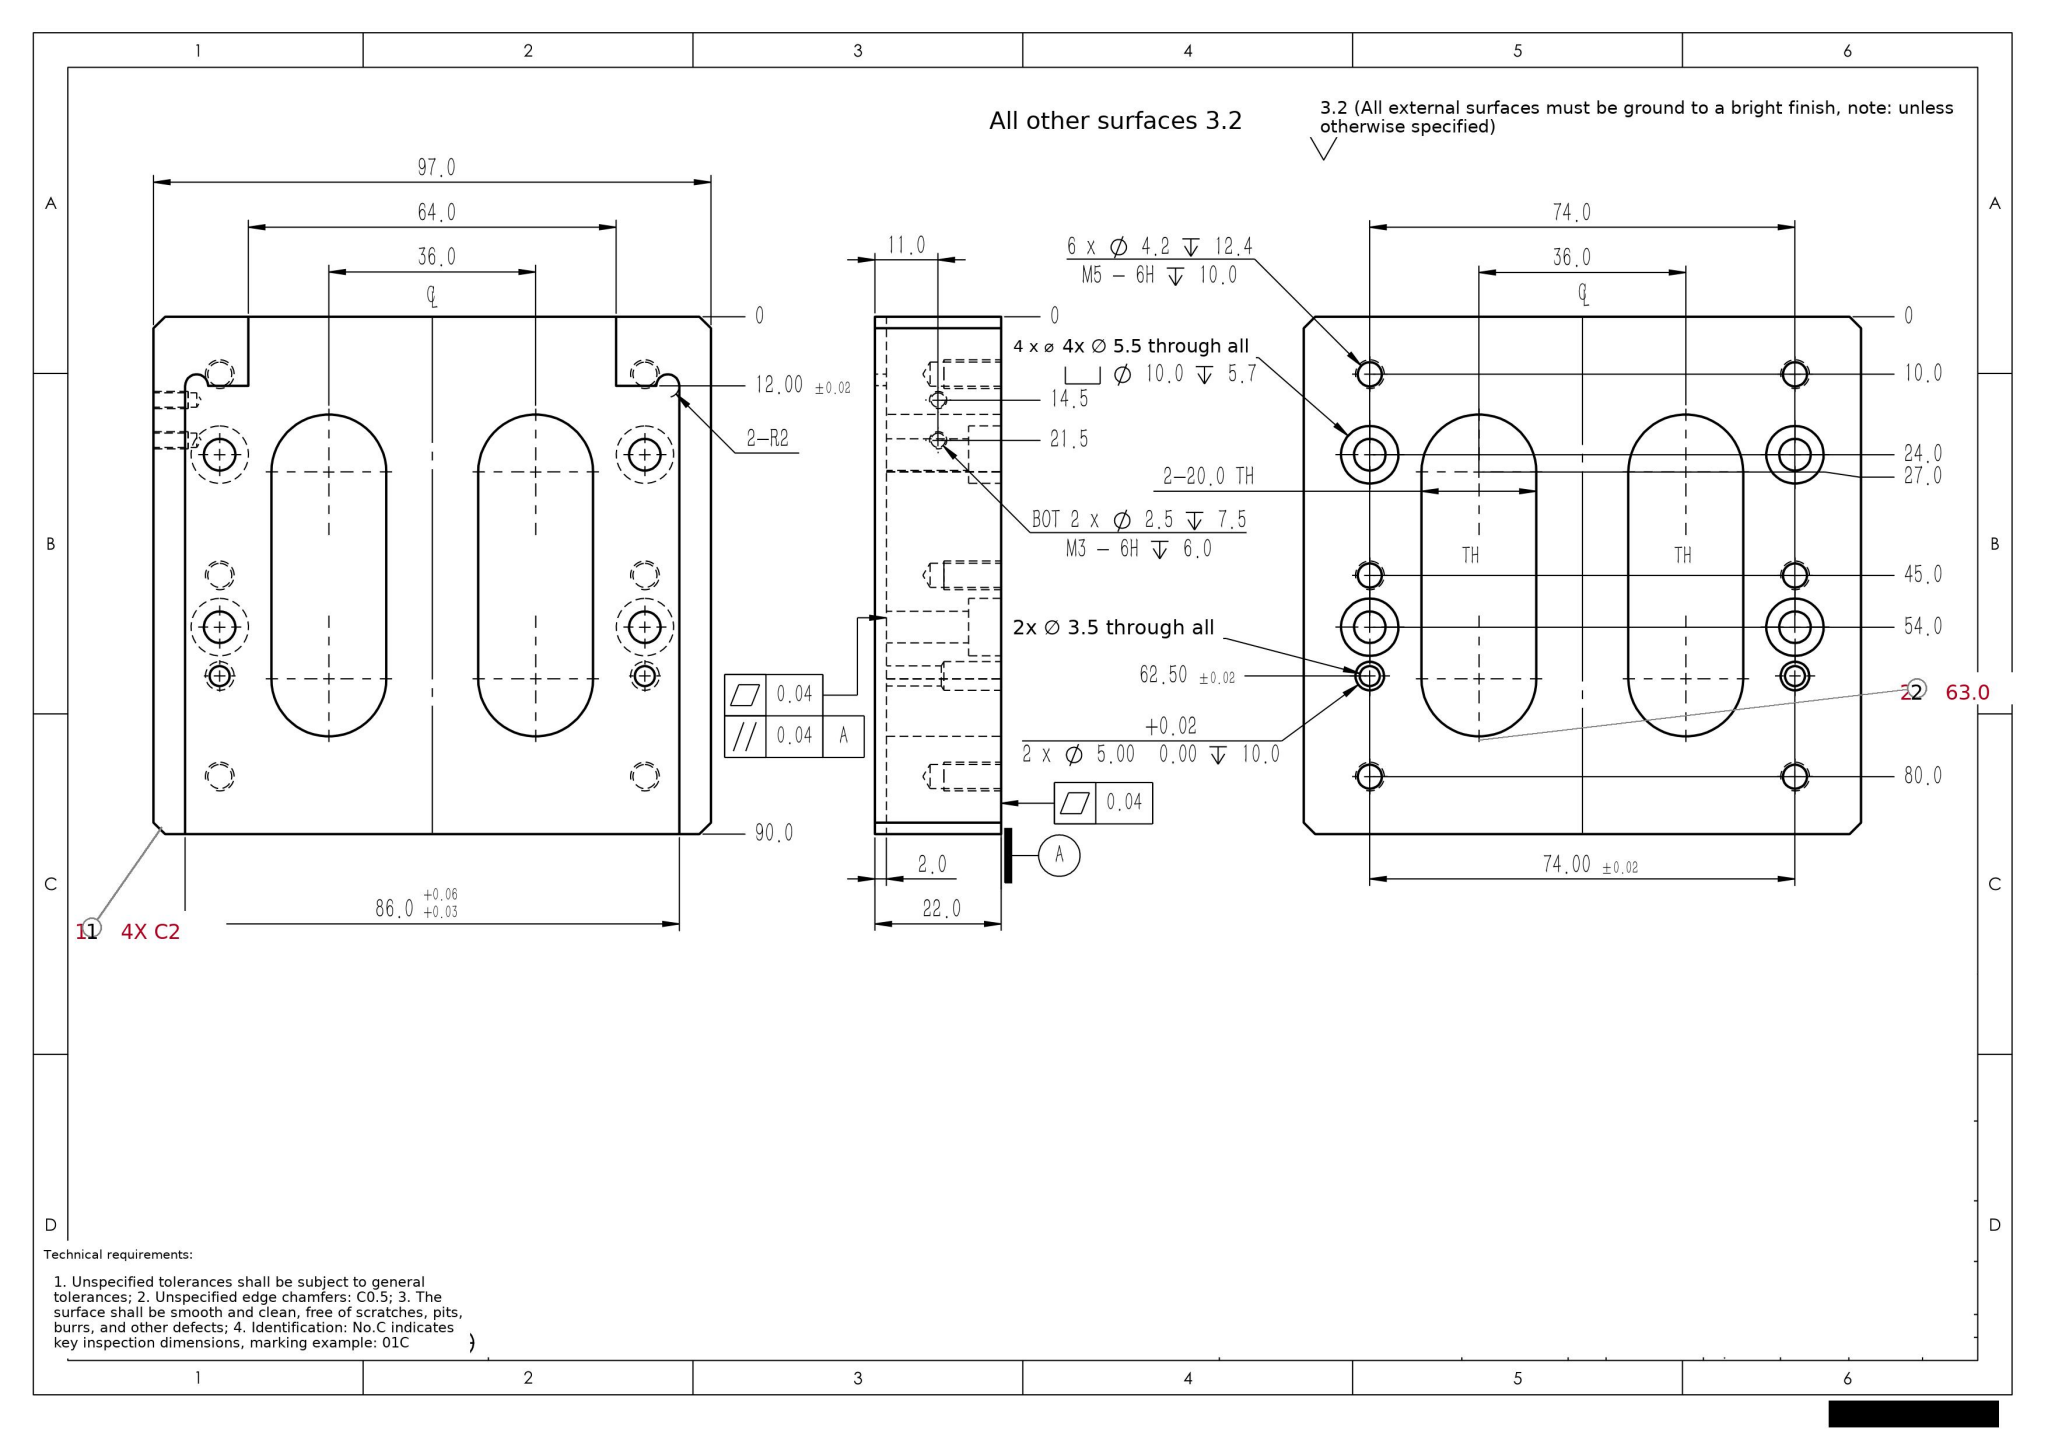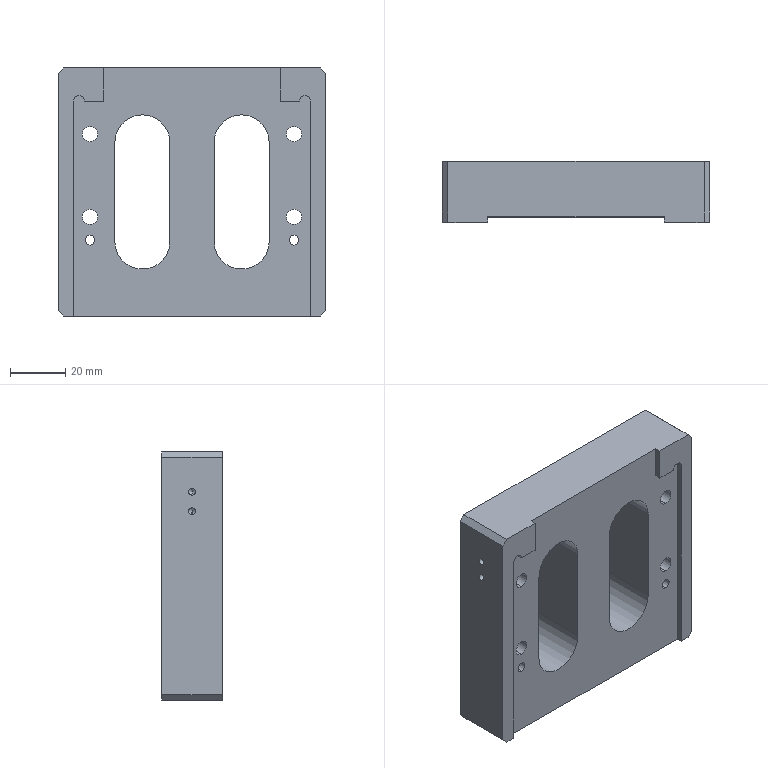Part | SolidWorks | mm | 1 solid | 96 faces | box 97 x 22 x 90 mm | volume 130660 mm3 | cylinder 50 | plane 26 | cone 20 | commonest cylinder face diameters 4.2 x12 10 x8 5.5 x8 20 x6 3.5 x4 2.5 x4 4 x4 5 x4
build123d program:
from build123d import *

# Parameters (mm, degrees)
SKETCH1_W                                         = 97
SKETCH1_H                                         = 90
BOSS_EXTRUDE1_DEPTH                               = 22
HOLE_SIZE_ACCORDING_TO_HEXAGON_SOCKET_D           = 5.5
HOLE_SIZE_ACCORDING_TO_HEXAGON_SOCKET_CBORE_D     = 10
HOLE_SIZE_ACCORDING_TO_HEXAGON_SOCKET_CBORE_DEPTH = 5.7
M5_TAPPED_HOLE1_D                                 = 4.2
M5_TAPPED_HOLE1_DEPTH                             = 12.4
M5_TAPPED_HOLE1_TIP                               = 1.262
SIZE_MM_DOWEL_PIN_HOLE2_D                         = 5
SIZE_MM_DOWEL_PIN_HOLE2_DEPTH                     = 10
SIZE_MM_DOWEL_PIN_HOLE2_TIP                       = 1.502
SKETCH15_W                                        = 86
SKETCH15_H                                        = 78
CUT_EXTRUDE4_DEPTH                                = 2
SKETCH18_W                                        = 64
SKETCH18_H                                        = 12
CUT_EXTRUDE9_DEPTH                                = 2
SKETCH16_R                                        = 2
CUT_EXTRUDE6_DEPTH                                = 2
CUT_EXTRUDE7_DEPTH                                = 70.723
M3_TAPPED_HOLE1_D                                 = 2.5
M3_TAPPED_HOLE1_DEPTH                             = 7.5
M3_TAPPED_HOLE1_TIP                               = 0.7511
F_3_5_3_5_DIAMETER_HOLE1_D                        = 3.5
CHAMFER1_SIZE                                     = 2


with BuildPart() as part:
    # Sketch1 → Boss-Extrude1 (new body)
    with BuildSketch(Plane(origin=(0, 0, 0), x_dir=(1, 0, 0), z_dir=(0, 1, 0))):
        Rectangle(SKETCH1_W, SKETCH1_H)
    extrude(amount=BOSS_EXTRUDE1_DEPTH)

    # Hole Size _ according to_ Hexagon Socket (through all)
    with Locations(Plane(origin=(0, 22, 0), x_dir=(1, 0, 0), z_dir=(0, 1, 0))):
        with Locations((-37, 9), (-37, -21), (37, -21), (37, 9)):
            CounterBoreHole(HOLE_SIZE_ACCORDING_TO_HEXAGON_SOCKET_D / 2, HOLE_SIZE_ACCORDING_TO_HEXAGON_SOCKET_CBORE_D / 2, HOLE_SIZE_ACCORDING_TO_HEXAGON_SOCKET_CBORE_DEPTH)

    # M5 Tapped Hole1
    with Locations(Plane(origin=(0, 22, 0), x_dir=(1, 0, 0), z_dir=(0, 1, 0))):
        with Locations((-37, -35), (-37, 0), (-37, 35), (37, 35), (37, 0), (37, -35)):
            Hole(M5_TAPPED_HOLE1_D / 2, depth=M5_TAPPED_HOLE1_DEPTH)
            with Locations((0, 0, -(M5_TAPPED_HOLE1_DEPTH + M5_TAPPED_HOLE1_TIP / 2))):  # 118° drill point
                Cone(0, M5_TAPPED_HOLE1_D / 2, M5_TAPPED_HOLE1_TIP, mode=Mode.SUBTRACT)

    # Size mm Dowel Pin Hole2
    with Locations(Plane(origin=(0, 22, 0), x_dir=(1, 0, 0), z_dir=(0, 1, 0))):
        with Locations((-37, 17.5), (37, 17.5)):
            Hole(SIZE_MM_DOWEL_PIN_HOLE2_D / 2, depth=SIZE_MM_DOWEL_PIN_HOLE2_DEPTH)
            with Locations((0, 0, -(SIZE_MM_DOWEL_PIN_HOLE2_DEPTH + SIZE_MM_DOWEL_PIN_HOLE2_TIP / 2))):  # 118° drill point
                Cone(0, SIZE_MM_DOWEL_PIN_HOLE2_D / 2, SIZE_MM_DOWEL_PIN_HOLE2_TIP, mode=Mode.SUBTRACT)

    # Sketch15 → Cut-Extrude4 (cut)
    with BuildSketch(Plane(origin=(0, 0, 0), x_dir=(-1, 0, 0), z_dir=(0, -1, 0))):
        with Locations((0, 6)):
            Rectangle(SKETCH15_W, SKETCH15_H)
    extrude(amount=-CUT_EXTRUDE4_DEPTH, mode=Mode.SUBTRACT)

    # Sketch18 → Cut-Extrude9 (cut)
    with BuildSketch(Plane(origin=(0, 2, 0), x_dir=(-1, 0, 0), z_dir=(0, -1, 0))):
        with Locations((0, -39)):
            Rectangle(SKETCH18_W, SKETCH18_H)
    extrude(amount=CUT_EXTRUDE9_DEPTH, mode=Mode.SUBTRACT)

    # Sketch16 → Cut-Extrude6 (cut)
    with BuildSketch(Plane.XZ.offset(-2)):
        with Locations((41, 33)):
            Circle(SKETCH16_R)
        with Locations((-41, 33)):
            Circle(SKETCH16_R)
    extrude(amount=CUT_EXTRUDE6_DEPTH, mode=Mode.SUBTRACT)

    # Sketch17 → Cut-Extrude7 (cut, through all)
    with BuildSketch(Plane(origin=(0, 22, 0), x_dir=(1, 0, 0), z_dir=(0, 1, 0))):
        with BuildLine():
            Line((8, -18), (8, 18))
            ThreePointArc((8, 18), (18, 28), (28, 18))
            Line((28, 18), (28, -18))
            ThreePointArc((28, -18), (18, -28), (8, -18))
        make_face()
        with BuildLine():
            Line((-28, -18), (-28, 18))
            ThreePointArc((-28, 18), (-18, 28), (-8, 18))
            Line((-8, 18), (-8, -18))
            ThreePointArc((-8, -18), (-18, -28), (-28, -18))
        make_face()
    extrude(amount=-CUT_EXTRUDE7_DEPTH, mode=Mode.SUBTRACT)

    # M3 Tapped Hole1
    with Locations(Plane.ZY.offset(48.5)):
        with Locations((30.5, 11), (23.5, 11)):
            Hole(M3_TAPPED_HOLE1_D / 2, depth=M3_TAPPED_HOLE1_DEPTH)
            with Locations((0, 0, -(M3_TAPPED_HOLE1_DEPTH + M3_TAPPED_HOLE1_TIP / 2))):  # 118° drill point
                Cone(0, M3_TAPPED_HOLE1_D / 2, M3_TAPPED_HOLE1_TIP, mode=Mode.SUBTRACT)

    # 3.5 _3.5_ Diameter Hole1 (through all)
    with Locations(Plane(origin=(0, 22, 0), x_dir=(1, 0, 0), z_dir=(0, 1, 0))):
        with Locations((37, 17.5), (-37, 17.5)):
            Hole(F_3_5_3_5_DIAMETER_HOLE1_D / 2)

    # Chamfer1
    chamfer1_edges = [part.edges().sort_by_distance(p)[0] for p in [
        (-48.5, 11, -45),
        (48.5, 11, -45),
        (48.5, 11, 45),
        (-48.5, 11, 45),
    ]]
    chamfer(chamfer1_edges, length=CHAMFER1_SIZE)


solid = part.part